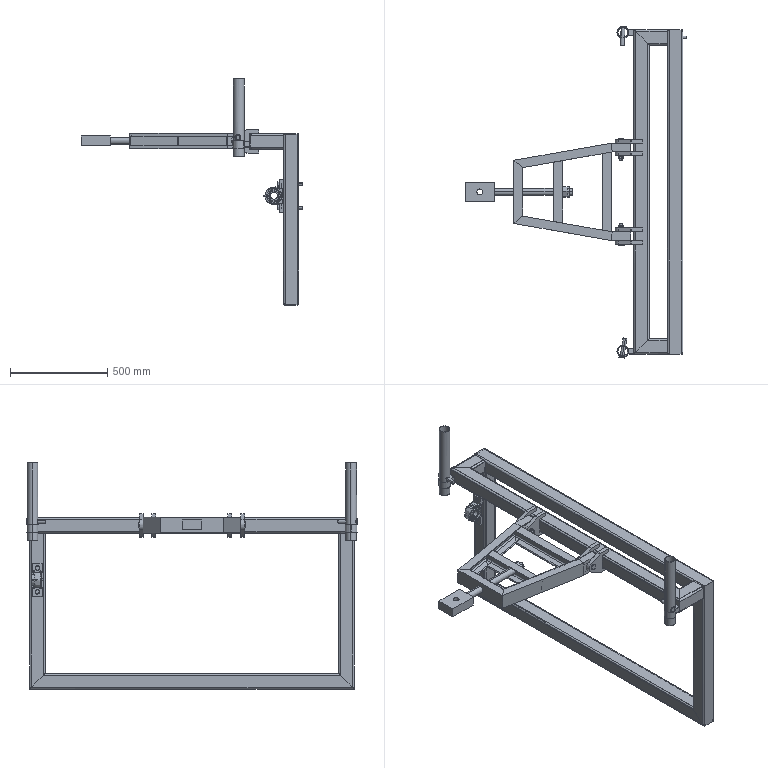Assembly | SolidWorks | mm | 21 component files | 33 solids | 778 faces | box 1137.45 x 1702.88 x 1160 mm | volume 14604811 mm3 | plane 399 | cylinder 250 | cone 78 | sphere 34 | torus 12 | spline 5 | commonest cylinder face diameters 20 x48 10 x28 16 x26 25 x16 8 x14 2.25 x12 30 x10 36 x8
Bill of materials:
6.1Frame | 1 |  | Flat rectangular frame of square-section bar. A second straight bar runs alongside the top member, so the top edge is a short open rectangle seen from above.
6TractionAxis | 1 |  | Rectangular block with one through hole, and a long round rod sticking out from one side face.
7LegTravel | 2 |  | Straight thin-walled round tube, open at both ends, with small cross holes through the wall near one end.
7TractionFrame | 1 |  | Ladder-like frame of thin formed channel members: two side channels joined by cross members, with a slightly tapered (trapezoidal) outline in plan view and holes in the webs.
7TractionPlate | 4 |  | Flat plate of even thickness with a rounded, tapering end carrying one round hole, and an open rectangular slot at the other end that forms a fork shape.
7TutorialFrame | 2 |  | Short thin-walled round ring (cylindrical sleeve) with a hollow square-section tube stub sticking out sideways from its outer wall.
7xiao | 2 | 45 | Headed cylindrical pin: a plain straight round shank with a short wider disc head at one end.
GB_T5785-2016[HexHeadBoltFineThread(M14_1.5)_120] | 2 |  | Hex-head bolt-like part: a hexagonal head with a round collar or washer face underneath, and a long, plain, straight cylindrical shank with a chamfered end.
GB_T6170-2015[Type1HexNutM16] | 2 |  | Hexagonal nut-like part with a large plain central bore, chamfered (curved) hex corners on one face, and a short round collar or washer face on the other side.
GB_T7810-2017[BearingWithVerticalHousing(UELP)UELP207] | 1 |  | Part that looks like a pillow-block bearing housing: a flat rectangular base with two elongated mounting holes in recessed pockets, and a rounded housing on top holding a ring-shaped insert with a central through bore. A small knob sticks out of the housing on the side opposite the base.
GB_T9459-1988[HexSlottedThinNutFineThreadM36_3] | 1 |  | Slotted (castle-style) hexagonal nut: a hex prism with chamfered ends and a central through bore. Six radial rectangular slots are cut across one end face, one slot through each hex flat.
ShaftDiameterToleranceOptionalTypeBHingePin[KPVHBH25-85] | 2 |  | Stepped cylindrical pin: a short head flange with a flat on it at one end, a long main shank, and a shorter, smaller-diameter spigot at the other end, with a small neck or groove at the step.
Mates:
1. concentric | 7TractionFrame-1 face at (133.529, 246.21, 600) dir (0, -1, 0) r 12.5 | 7TractionPlate-2 face at (133.529, -273.79, 600) dir (0, 1, 0) r 12.5
2. coincident | 7TractionFrame-1 face at (83.529, -253.79, 560) dir (0, -1, 0) | 7TractionPlate-2 face at (213.102, -253.79, 608.582) dir (0, 1, 0)
3. concentric | 7TractionFrame-1 face at (133.529, 246.21, 600) dir (0, -1, 0) r 12.5 | 7TractionPlate-1 face at (133.529, -208.79, 600) dir (0, 1, 0) r 12.5
4. coincident | 7TractionFrame-1 face at (83.529, -208.79, 560) dir (0, 1, 0) | 7TractionPlate-1 face at (213.102, -208.79, 608.582) dir (0, -1, 0)
5. concentric | 7TractionFrame-1 face at (133.529, 246.21, 600) dir (0, -1, 0) r 12.5 | 7TractionPlate-3 face at (133.529, 246.21, 600) dir (0, 1, 0) r 12.5
6. concentric | 7TractionPlate-3 face at (133.529, 246.21, 600) dir (0, 1, 0) r 12.5 | 7TractionPlate-4 face at (133.529, 181.21, 600) dir (0, 1, 0) r 12.5
7. coincident | 7TractionFrame-1 face at (183.529, 201.21, 560) dir (0, -1, 0) | 7TractionPlate-4 face at (213.102, 201.21, 608.582) dir (0, 1, 0)
8. parallel | 7TractionFrame-1 face at (183.529, 201.21, 640) dir (0, 0, 1) | 7TractionPlate-4 face at (213.102, 181.21, 657.679) dir (0, 0, 1)
9. parallel | 7TractionFrame-1 face at (183.529, 201.21, 640) dir (0, 0, 1) | 7TractionPlate-3 face at (213.102, 246.21, 657.679) dir (0, 0, 1)
10. parallel | 7TractionFrame-1 face at (83.529, -208.79, 640) dir (0, 0, 1) | 7TractionPlate-2 face at (213.102, -273.79, 657.679) dir (0, 0, 1)
11. parallel | 7TractionFrame-1 face at (83.529, -208.79, 640) dir (0, 0, 1) | 7TractionPlate-1 face at (213.102, -208.79, 657.679) dir (0, 0, 1)
12. concentric | 7TractionPlate-1 face at (133.529, -208.79, 600) dir (0, 1, 0) r 12.5 | ShaftDiameterToleranceOptionalTypeBHingePin[KPVHBH25-85]-1 face at (133.529, -278.79, 600) dir (0, -1, 0) r 12.5
13. coincident | 7TractionPlate-2 face at (213.102, -273.79, 608.582) dir (0, -1, 0) | ShaftDiameterToleranceOptionalTypeBHingePin[KPVHBH25-85]-1 face at (139.257, -273.79, 613.863) dir (0, 1, 0)
14. concentric | ShaftDiameterToleranceOptionalTypeBHingePin[KPVHBH25-85]-1 face at (133.529, -278.79, 600) dir (0, -1, 0) r 8 | GB_T6170-2015[Type1HexNutM16]-1 face at (133.529, -188.79, 600) dir (0, 1, 0) r 8
15. coincident | ShaftDiameterToleranceOptionalTypeBHingePin[KPVHBH25-85]-1 face at (138.302, -188.79, 611.553) dir (0, 1, 0) | GB_T6170-2015[Type1HexNutM16]-1 face at (147.386, -188.79, 600) dir (0, -1, 0)
16. concentric | 7TractionPlate-3 face at (133.529, 246.21, 600) dir (0, 1, 0) r 12.5 | ShaftDiameterToleranceOptionalTypeBHingePin[KPVHBH25-85]-2 face at (133.529, 271.21, 600) dir (0, 1, 0) r 12.5
17. coincident | 7TractionPlate-3 face at (213.102, 266.21, 608.582) dir (0, 1, 0) | ShaftDiameterToleranceOptionalTypeBHingePin[KPVHBH25-85]-2 face at (148.529, 266.21, 600) dir (0, -1, 0)
18. concentric | ShaftDiameterToleranceOptionalTypeBHingePin[KPVHBH25-85]-2 face at (133.529, 271.21, 600) dir (0, 1, 0) r 8 | GB_T6170-2015[Type1HexNutM16]-2 face at (133.529, 166.41, 600) dir (0, 1, 0) r 8
19. coincident | ShaftDiameterToleranceOptionalTypeBHingePin[KPVHBH25-85]-2 face at (146.029, 181.21, 600) dir (0, -1, 0) | GB_T6170-2015[Type1HexNutM16]-2 face at (147.386, 181.21, 600) dir (0, 1, 0)
20. concentric | 7TractionFrame-1 face at (-115.559, -3.79, 600) dir (-1, 0, 0) r 18 | 6TractionAxis-1 face at (-116.471, -3.79, 600) dir (-1, 0, 0) r 18
21. distance | 6TractionAxis-1 face at (-516.471, -3.79, 600) dir (1, 0, 0) | 7TractionFrame-1 face at (-416.471, 158.046, 560) dir (-1, 0, 0)
22. parallel | 7TractionFrame-1 face at (-371.471, 158.046, 560) dir (0, 0, -1) | 6TractionAxis-1 face at (-666.471, -53.79, 575) dir (0, 0, -1)
23. coincident | 7TractionFrame-1 face at (-166.471, -209.709, 560) dir (1, 0, 0) | GB_T9459-1988[HexSlottedThinNutFineThreadM36_3]-1 face at (-166.471, -34.07, 556.934) dir (-1, 0, 0)
24. concentric | 6TractionAxis-1 face at (-116.471, -3.79, 600) dir (-1, 0, 0) r 18 | GB_T9459-1988[HexSlottedThinNutFineThreadM36_3]-1 face at (-131.771, -3.79, 600) dir (-1, 0, 0) r 18
25. distance | 7TractionPlate-3 face at (213.102, 266.21, 608.582) dir (0, 1, 0) | 6.1Frame-1 face at (238.48, 828.71, 567.679) dir (0, 1, 0)
26. coincident | 6.1Frame-1 face at (268.48, -796.29, 637.679) dir (0, 0, 1) | 7TractionPlate-3 face at (213.102, 246.21, 637.679) dir (0, 0, -1)
27. coincident | 6.1Frame-1 face at (198.48, -796.29, 567.679) dir (-1, 0, 0) | 7TractionPlate-3 face at (198.48, 246.21, 608.582) dir (1, 0, 0)
28. coincident | 6.1Frame-1 face at (198.48, -796.29, 567.679) dir (-1, 0, 0) | 7TutorialFrame-1 face at (198.48, -821.29, 597.679) dir (1, 0, 0)
29. coincident | 6.1Frame-1 edge at (198.48, -836.29, 567.679) dir (0, 1, 0) | 7TutorialFrame-1 face at (142.5, -821.29, 567.679) dir (0, 0, -1)
30. coincident | 6.1Frame-1 edge at (198.48, -836.29, 627.679) dir (0, 0, -1) | 7TutorialFrame-1 face at (142.5, -836.29, 597.679) dir (0, -1, 0)
31. concentric | 7TutorialFrame-1 face at (142.5, -821.29, 602.679) dir (0, 0, -1) r 27.5 | 7LegTravel-1 face at (142.5, -821.29, 517.679) dir (0, 0, 1) r 27.5
32. tangent | 7TutorialFrame-1 face at (142.5, -821.29, 602.679) dir (0, 0, 1) | 7xiao-1 face at (137.838, -848.392, 617.679) dir (-0.1695, -0.9855, 0) r 15
33. concentric | 7LegTravel-1 face at (106.052, -1033.179, 617.679) dir (0.1695, 0.9855, 0) r 10 | 7xiao-1 face at (153.942, -754.767, 617.679) dir (-0.1695, -0.9855, 0) r 10
34. tangent | 7LegTravel-1 face at (142.5, -821.29, 517.679) dir (0, 0, 1) r 27.5 | 7xiao-1 face at (137.838, -848.392, 617.679) dir (0.1695, 0.9855, 0)
35. coincident | 6.1Frame-1 face at (198.48, -796.29, 567.679) dir (-1, 0, 0) | 7TutorialFrame-2 face at (198.48, 813.71, 597.679) dir (1, 0, 0)
36. coincident | 6.1Frame-1 face at (238.48, 828.71, 567.679) dir (0, 1, 0) | 7TutorialFrame-2 face at (142.5, 828.71, 597.679) dir (0, 1, 0)
37. coincident | 6.1Frame-1 edge at (198.48, -836.29, 567.679) dir (0, 1, 0) | 7TutorialFrame-2 edge at (198.48, 828.71, 567.679) dir (0, -1, 0)
38. concentric | 7TutorialFrame-2 face at (142.5, 813.71, 602.679) dir (0, 0, -1) r 27.5 | 7LegTravel-2 face at (142.5, 813.71, 517.679) dir (0, 0, 1) r 27.5
39. tangent | 7TutorialFrame-2 face at (142.5, 813.71, 602.679) dir (0, 0, 1) | 7xiao-2 face at (144.079, 841.164, 617.679) dir (0.05742, 0.9983, 0) r 15
40. concentric | 7LegTravel-2 face at (130.154, 599.064, 617.679) dir (0.05742, 0.9983, 0) r 10 | 7xiao-2 face at (138.624, 746.321, 617.679) dir (0.05742, 0.9983, 0) r 10
41. tangent | 7LegTravel-2 face at (142.5, 813.71, 517.679) dir (0, 0, 1) r 27.5 | 7xiao-2 face at (144.079, 841.164, 617.679) dir (-0.05742, -0.9983, 0)
42. coincident | 6.1Frame-1 face at (370.98, 818.71, 597.679) dir (-1, 0, 0) | GB_T7810-2017[BearingWithVerticalHousing(UELP)UELP207]-1 face at (370.98, 812.71, 280.211) dir (1, 0, 0)
43. distance | GB_T7810-2017[BearingWithVerticalHousing(UELP)UELP207]-1 face at (353.98, 764.71, 277.211) dir (0, -1, 0) | 6.1Frame-1 face at (440.98, 748.71, 597.679) dir (0, -1, 0)
44. concentric | GB_T7810-2017[BearingWithVerticalHousing(UELP)UELP207]-1 face at (269.513, 788.71, 257.179) dir (1, 0, 0) r 8 | GB_T5785-2016[HexHeadBoltFineThread(M14_1.5)_120]-1 face at (342.18, 788.71, 257.179) dir (-1, 0, 0) r 7
45. coincident | GB_T7810-2017[BearingWithVerticalHousing(UELP)UELP207]-1 face at (350.98, 812.71, 277.211) dir (-1, 0, 0) | GB_T5785-2016[HexHeadBoltFineThread(M14_1.5)_120]-1 face at (350.98, 800.326, 253.707) dir (1, 0, 0)
46. concentric | GB_T7810-2017[BearingWithVerticalHousing(UELP)UELP207]-1 face at (269.513, 788.71, 378.179) dir (1, 0, 0) r 8 | GB_T5785-2016[HexHeadBoltFineThread(M14_1.5)_120]-2 face at (342.18, 788.71, 378.179) dir (-1, 0, 0) r 7
47. coincident | GB_T7810-2017[BearingWithVerticalHousing(UELP)UELP207]-1 face at (350.98, 812.71, 400.679) dir (-1, 0, 0) | GB_T5785-2016[HexHeadBoltFineThread(M14_1.5)_120]-2 edge at (350.98, 788.71, 378.179) dir (-1, 0, 0) r 7.6